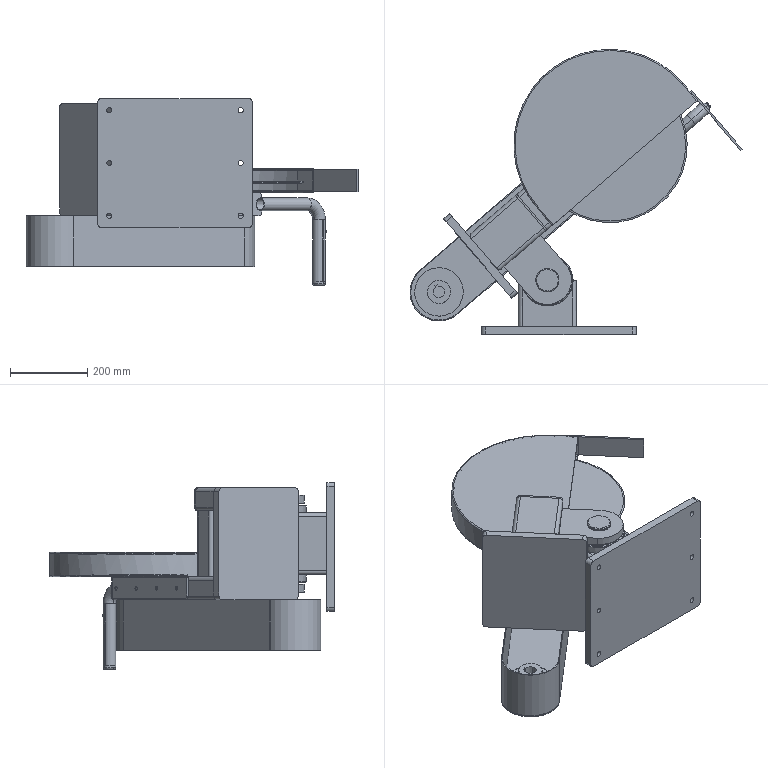Assembly | SolidWorks | mm | 14 component files | 27 solids | 1396 faces | box 858.55 x 737.31 x 483.5 mm | volume 12580641 mm3 | sphere 448 | cylinder 337 | plane 308 | torus 228 | cone 72 | spline 3 | commonest cylinder face diameters 20 x41 9.5 x24 10 x20 30 x18 103.5 x16 60 x16 49.5 x16 125.5 x16
Bill of materials:
BeltGuard | 1 | Stainless Steel | Solid obround (stadium-shaped) bar: a straight prism with two fully rounded ends and flat parallel top and bottom faces. Shape resembles a rounded-end parallel key.
CuttingAxis | 1 | Stainless Steel | Stepped cylindrical shaft with a circular flange at one end. The flange has four through holes evenly spaced on a bolt circle and a small raised central boss with a small center recess. Below the flange the shaft has three sections: a short larger collar, a long middle section and a smaller-diameter end section.
CuttingMachineFrame | 1 | Stainless Steel | Bracket with a thin flat base plate and a block-like body with two projecting tabs that have rounded ends and through holes, forming a clevis-like pair. A long flat rectangular arm extends sideways and ends in a through hole with a raised ring or counterbore.
CuttingMachineRotaryBase | 1 | Stainless Steel | Rectangular mounting plate with rounded corners and six small through holes, three along each of two opposite edges. A web or standoff on one face carries a hollow open-ended cylindrical tube whose axis runs parallel to the plate.
GB_T276-94DeepGrooveBallBearing6015-2RZ | 2 | GCr4 | Annular assembly-like ring with concentric inner and outer rings separated by a gap containing a circle of evenly spaced rolling elements. The geometry resembles an open radial ball bearing.
GB_T276-94DeepGrooveBallBearing61907-2RZ | 2 | GCr4 | Annular ring assembly very similar to the previous ring part: inner and outer rings with a circle of evenly spaced rolling elements in the gap between them, resembling an open radial ball bearing. Proportions differ slightly, with a somewhat thicker cross-section relative to the bore.
Handle | 1 | Stainless Steel | Round tube or rod bent 90 degrees. One end joins a small rectangular flat plate with two small through holes; at that end the tube looks hollow with an open bore. The other leg ends with rounded edges and has a small cylindrical stub or pin on its side, and possibly a small stub at the tip.
RotationAxisB | 1 | Stainless Steel | Stepped cylindrical pin with a larger central body and shorter reduced-diameter journals at both ends. Each journal has a narrow groove near its end, and the ends are slightly chamfered.
SawBlade | 1 | 45 | Thin flat circular disc with a central round hole and four smaller holes evenly spaced on a bolt circle around it. The outer edge appears tapered or beveled to a thin edge.
SawBladeGuardB | 1 | Stainless Steel | Sheet-metal style cover: a roughly semicircular flat top panel with downturned flanges along its straight edge. The flanges are stepped or offset and carry rows of small through holes. A thin flange projects at one end.
SmallPulley | 2 |  | Multi-groove pulley (sheave) with three V-profile grooves and an extended cylindrical hub on one side. The central bore has a single keyway.
Mates:
1. concentric | CuttingMachineRotaryBase-1 face at (-534.67, 967.452, 350.7) dir (0, 0, -1) r 57.5 | GB_T276-94DeepGrooveBallBearing6015-2RZ-1 face at (-534.67, 967.452, 330.7) dir (0, 0, 1) r 57.5
2. coincident | CuttingMachineRotaryBase-1 face at (-534.67, 967.452, 320.7) dir (0, 0, 1) | GB_T276-94DeepGrooveBallBearing6015-2RZ-1 face at (-513.066, 915.354, 320.7) dir (0, 0, -1)
3. coincident | CuttingMachineRotaryBase-1 face at (-534.67, 967.452, 180.7) dir (0, 0, -1) | GB_T276-94DeepGrooveBallBearing6015-2RZ-2 face at (-513.066, 915.354, 180.7) dir (0, 0, 1)
4. concentric | CuttingMachineRotaryBase-1 face at (-534.67, 967.452, 350.7) dir (0, 0, -1) r 57.5 | GB_T276-94DeepGrooveBallBearing6015-2RZ-2 face at (-534.67, 967.452, 170.7) dir (0, 0, -1) r 57.5
5. concentric | GB_T276-94DeepGrooveBallBearing6015-2RZ-2 face at (-534.67, 967.452, 158.279) dir (0, 0, -1) r 37.5 | RotationAxisB-1 face at (-534.67, 967.452, 382.9) dir (0, 0, 1) r 37.5
6. width | GB_T276-94DeepGrooveBallBearing6015-2RZ-2 face at (-517.816, 926.808, 160.7) dir (0, 0, -1) | GB_T276-94DeepGrooveBallBearing6015-2RZ-1 face at (-517.816, 926.808, 340.7) dir (0, 0, 1) | RotationAxisB-1 face at (-523.179, 939.741, 355.7) dir (0, 0, 1) | RotationAxisB-1 face at (-520.306, 932.813, 145.7) dir (0, 0, -1)
7. width | RotationAxisB-1 face at (-523.179, 939.741, 355.7) dir (0, 0, 1) | RotationAxisB-1 face at (-520.306, 932.813, 145.7) dir (0, 0, -1) | CuttingMachineFrame-1 face at (-534.67, 967.452, 355.7) dir (0, 0, -1) | CuttingMachineFrame-1 face at (-534.67, 967.452, 145.7) dir (0, 0, 1)
8. concentric | CuttingMachineFrame-1 face at (-373.165, 1316.761, 281.766) dir (0, 0, -1) r 27.5 | GB_T276-94DeepGrooveBallBearing61907-2RZ-1 face at (-373.165, 1316.761, 115.7) dir (0, 0, 1) r 27.5
9. distance | GB_T276-94DeepGrooveBallBearing61907-2RZ-1 face at (-373.165, 1343.661, 110.7) dir (0, 0, -1) | CuttingMachineFrame-1 face at (-373.165, 1316.761, 100.7) dir (0, 0, -1)
10. concentric | CuttingMachineFrame-1 face at (-373.165, 1316.761, 281.766) dir (0, 0, -1) r 27.5 | GB_T276-94DeepGrooveBallBearing61907-2RZ-2 face at (-373.165, 1316.761, 155.7) dir (0, 0, 1) r 27.5
11. distance | GB_T276-94DeepGrooveBallBearing61907-2RZ-2 face at (-373.165, 1343.661, 160.7) dir (0, 0, 1) | CuttingMachineFrame-1 face at (-302.661, 1311.359, 170.7) dir (0, 0, 1)
12. concentric | GB_T276-94DeepGrooveBallBearing61907-2RZ-2 face at (-373.165, 1316.761, 168.121) dir (0, 0, 1) r 17.5 | CuttingAxis-1 face at (-373.165, 1316.761, 195.1) dir (0, 0, 1) r 17.5
13. coincident | GB_T276-94DeepGrooveBallBearing61907-2RZ-2 face at (-373.165, 1337.311, 160.7) dir (0, 0, 1) | CuttingAxis-1 face at (-380.826, 1335.235, 160.7) dir (0, 0, -1)
14. concentric | CuttingAxis-1 face at (-373.165, 1316.761, 195.1) dir (0, 0, 1) r 15 | SawBlade-1 face at (-373.165, 1316.761, 194.9) dir (0, 0, -1) r 15
15. coincident | CuttingAxis-1 face at (-378.911, 1330.617, 190.7) dir (0, 0, 1) | SawBlade-1 face at (-373.165, 1316.761, 190.7) dir (0, 0, -1)
16. concentric | CuttingAxis-1 face at (-388.487, 1353.71, 190.7) dir (0, 0, 1) r 3.4 | SawBlade-1 face at (-388.487, 1353.71, 190.699) dir (0, 0, 1) r 4.75
17. coincident | CuttingMachineFrame-1 face at (-374.274, 1394.855, 115.7) dir (-0.651, 0.7591, 0) | SawBladeGuardB-1 face at (-366.684, 1401.366, 228.701) dir (0.651, -0.7591, 0)
18. coincident | CuttingMachineFrame-1 face at (-360.174, 1393.775, 115.7) dir (0.7591, 0.651, 0) | SawBladeGuardB-1 face at (-288.561, 1310.279, 228.701) dir (-0.7591, -0.651, 0)
19. coincident | CuttingMachineFrame-1 face at (-302.661, 1311.359, 165.7) dir (0, 0, 1) | SawBladeGuardB-1 face at (-373.165, 1316.761, 165.7) dir (0, 0, -1)
20. concentric | RotationAxisB-1 face at (-534.67, 967.452, 382.9) dir (0, 0, 1) r 30 | CuttingMachineFrame-1 face at (-534.67, 967.452, 145.7) dir (0, 0, -1) r 30
21. concentric | CuttingAxis-1 face at (-373.165, 1316.761, 195.1) dir (0, 0, 1) r 15 | SmallPulley-1 face at (-373.165, 1316.761, -11.2) dir (0, 0, -1) r 15
22. coincident | SmallPulley-1 face at (-373.131, 1331.761, -11.2) dir (0, 0, -1) | SmallPulley-2 face at (-820.681, 951.719, -11.2) dir (0, 0, -1)
23. concentric | CuttingAxis-1 face at (-373.165, 1316.761, 195.1) dir (0, 0, 1) r 17.5 | BeltGuard-1 face at (-373.165, 1316.761, 105.7) dir (0, 0, -1) r 73
24. concentric | SmallPulley-2 face at (-814.935, 937.863, -11.2) dir (0, 0, -1) r 51.3 | BeltGuard-1 face at (-814.935, 937.863, 105.7) dir (0, 0, -1) r 75
25. coincident | CuttingMachineFrame-1 face at (-367.764, 1387.265, 105.7) dir (0, 0, -1) | BeltGuard-1 face at (-814.935, 937.863, 105.7) dir (0, 0, 1)
26. coincident | CuttingMachineFrame-1 face at (-296.151, 1303.769, 155.7) dir (0.651, -0.7591, 0) | Handle-1 face at (-331.827, 1273.17, 135.7) dir (-0.651, 0.7591, 0)
27. coincident | CuttingMachineFrame-1 face at (-302.661, 1311.359, 165.7) dir (0, 0, 1) | Handle-1 face at (-286.283, 1312.232, 165.7) dir (0, 0, 1)
28. coincident | SawBladeGuardB-1 face at (-366.36, 1405.596, 105.7) dir (0.7591, 0.651, 0) | Handle-1 face at (-286.283, 1312.232, 105.7) dir (0.7591, 0.651, 0)